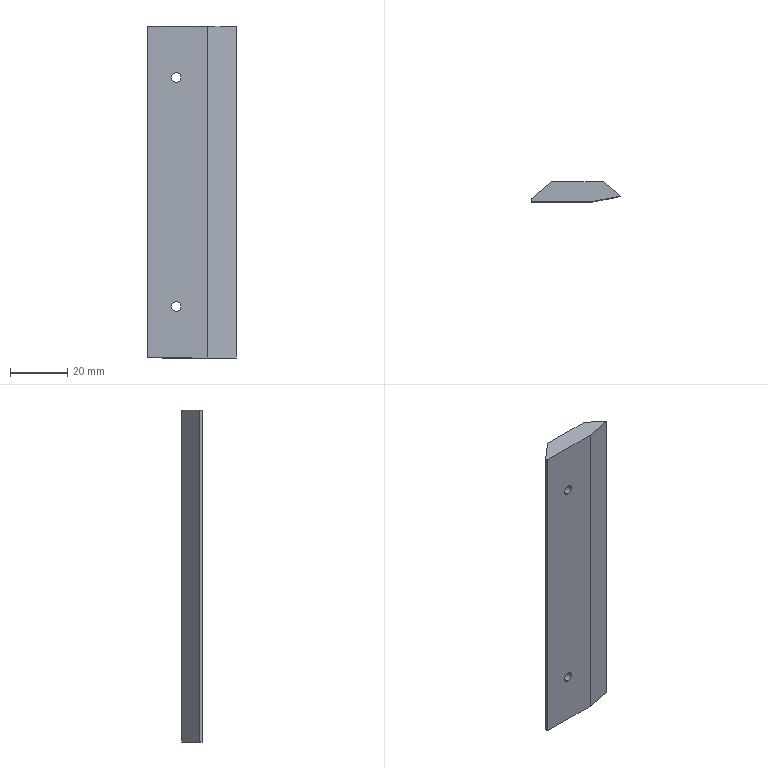Component | SolidWorks | 121.1-1 | 1 solid | 12 faces | box 31 x 7 x 116 mm | volume 19716 mm3 | plane 8 | cylinder 4 | commonest cylinder face diameters 3.3 x4
build123d program:
from build123d import *

# Parameters (mm, degrees)
BOSS_EXTRUDE1_DEPTH   = 58
M4_TAPPED_HOLE1_D     = 3.3
M4_TAPPED_HOLE1_DEPTH = 80
M4_TAPPED_HOLE1_TIP   = 0.9914


with BuildPart() as part:
    # Sketch1 → Boss-Extrude1 (new, symmetric)
    with BuildSketch(Plane.XY):
        Polygon((0, 0), (21, 0), (21, 1), (14, 7), (-4, 7), (-10, 2), align=None)
    extrude(amount=BOSS_EXTRUDE1_DEPTH, both=True)

    # M4 Tapped Hole1
    with Locations(Plane(origin=(0, 7, 0), x_dir=(-1, 0, 0), z_dir=(0, 1, 0))):
        with Locations((-11, 40), (-11, -40)):
            Hole(M4_TAPPED_HOLE1_D / 2, depth=M4_TAPPED_HOLE1_DEPTH)
            with Locations((0, 0, -(M4_TAPPED_HOLE1_DEPTH + M4_TAPPED_HOLE1_TIP / 2))):  # 118° drill point
                Cone(0, M4_TAPPED_HOLE1_D / 2, M4_TAPPED_HOLE1_TIP, mode=Mode.SUBTRACT)


solid = part.part

# Placed as in the assembly
solid = solid.moved(Location((19, 152.5, 0), (-180, 0, 180)))
STEP:
#1=COLOUR_RGB('',0.7922,0.8196,0.9333);
#2=FILL_AREA_STYLE_COLOUR('',#1);
#3=FILL_AREA_STYLE('',(#2));
#4=SURFACE_STYLE_FILL_AREA(#3);
#5=SURFACE_SIDE_STYLE('',(#4));
#6=SURFACE_STYLE_USAGE(.BOTH.,#5);
#7=PRESENTATION_STYLE_ASSIGNMENT((#6));
#8=CARTESIAN_POINT('',(0.315,6.004,-1.51));
#9=VERTEX_POINT('',#8);
#10=CARTESIAN_POINT('',(0.315,6.004,-1.64));
#11=VERTEX_POINT('',#10);
#12=CARTESIAN_POINT('',(0.315,6.004,-1.575));
#13=DIRECTION('',(0.,1.,0.));
#14=DIRECTION('',(-0.,0.,-1.));
#15=AXIS2_PLACEMENT_3D('',#12,#13,#14);
#16=CIRCLE('',#15,0.06496);
#17=EDGE_CURVE('',#9,#11,#16,.T.);
#18=ORIENTED_EDGE('',*,*,#17,.F.);
#19=CARTESIAN_POINT('',(0.315,6.28,-1.51));
#20=VERTEX_POINT('',#19);
#21=CARTESIAN_POINT('',(0.315,6.28,-1.51));
#22=DIRECTION('',(0.,1.,0.));
#23=VECTOR('',#22,39.37);
#24=LINE('',#21,#23);
#25=EDGE_CURVE('',#9,#20,#24,.T.);
#26=ORIENTED_EDGE('',*,*,#25,.T.);
#27=CARTESIAN_POINT('',(0.315,6.28,-1.64));
#28=VERTEX_POINT('',#27);
#29=CARTESIAN_POINT('',(0.315,6.28,-1.575));
#30=DIRECTION('',(0.,1.,0.));
#31=DIRECTION('',(-0.,0.,-1.));
#32=AXIS2_PLACEMENT_3D('',#29,#30,#31);
#33=CIRCLE('',#32,0.06496);
#34=EDGE_CURVE('',#20,#28,#33,.T.);
#35=ORIENTED_EDGE('',*,*,#34,.T.);
#36=CARTESIAN_POINT('',(0.315,6.28,-1.64));
#37=DIRECTION('',(0.,1.,0.));
#38=VECTOR('',#37,39.37);
#39=LINE('',#36,#38);
#40=EDGE_CURVE('',#11,#28,#39,.T.);
#41=ORIENTED_EDGE('',*,*,#40,.F.);
#42=EDGE_LOOP('',(#18,#26,#35,#41));
#43=FACE_OUTER_BOUND('',#42,.T.);
#44=CARTESIAN_POINT('',(0.315,6.28,-1.575));
#45=DIRECTION('',(0.,1.,0.));
#46=DIRECTION('',(-0.,0.,-1.));
#47=AXIS2_PLACEMENT_3D('',#44,#45,#46);
#48=CYLINDRICAL_SURFACE('',#47,0.06496);
#49=ADVANCED_FACE('',(#43),#48,.F.);
#50=CARTESIAN_POINT('',(0.315,6.004,1.64));
#51=VERTEX_POINT('',#50);
#52=CARTESIAN_POINT('',(0.315,6.004,1.51));
#53=VERTEX_POINT('',#52);
#54=CARTESIAN_POINT('',(0.315,6.004,1.575));
#55=DIRECTION('',(0.,1.,0.));
#56=DIRECTION('',(-0.,0.,-1.));
#57=AXIS2_PLACEMENT_3D('',#54,#55,#56);
#58=CIRCLE('',#57,0.06496);
#59=EDGE_CURVE('',#51,#53,#58,.T.);
#60=ORIENTED_EDGE('',*,*,#59,.F.);
#61=CARTESIAN_POINT('',(0.315,6.28,1.64));
#62=VERTEX_POINT('',#61);
#63=CARTESIAN_POINT('',(0.315,6.28,1.64));
#64=DIRECTION('',(0.,1.,0.));
#65=VECTOR('',#64,39.37);
#66=LINE('',#63,#65);
#67=EDGE_CURVE('',#51,#62,#66,.T.);
#68=ORIENTED_EDGE('',*,*,#67,.T.);
#69=CARTESIAN_POINT('',(0.315,6.28,1.51));
#70=VERTEX_POINT('',#69);
#71=CARTESIAN_POINT('',(0.315,6.28,1.575));
#72=DIRECTION('',(0.,1.,0.));
#73=DIRECTION('',(-0.,0.,-1.));
#74=AXIS2_PLACEMENT_3D('',#71,#72,#73);
#75=CIRCLE('',#74,0.06496);
#76=EDGE_CURVE('',#62,#70,#75,.T.);
#77=ORIENTED_EDGE('',*,*,#76,.T.);
#78=CARTESIAN_POINT('',(0.315,6.28,1.51));
#79=DIRECTION('',(0.,1.,0.));
#80=VECTOR('',#79,39.37);
#81=LINE('',#78,#80);
#82=EDGE_CURVE('',#53,#70,#81,.T.);
#83=ORIENTED_EDGE('',*,*,#82,.F.);
#84=EDGE_LOOP('',(#60,#68,#77,#83));
#85=FACE_OUTER_BOUND('',#84,.T.);
#86=CARTESIAN_POINT('',(0.315,6.28,1.575));
#87=DIRECTION('',(0.,1.,0.));
#88=DIRECTION('',(-0.,0.,-1.));
#89=AXIS2_PLACEMENT_3D('',#86,#87,#88);
#90=CYLINDRICAL_SURFACE('',#89,0.06496);
#91=ADVANCED_FACE('',(#85),#90,.F.);
#92=CARTESIAN_POINT('',(1.142,6.083,2.283));
#93=VERTEX_POINT('',#92);
#94=CARTESIAN_POINT('',(0.748,6.004,2.283));
#95=VERTEX_POINT('',#94);
#96=CARTESIAN_POINT('',(1.142,6.083,2.283));
#97=DIRECTION('',(-0.9806,-0.1961,0.));
#98=VECTOR('',#97,39.37);
#99=LINE('',#96,#98);
#100=EDGE_CURVE('',#93,#95,#99,.T.);
#101=ORIENTED_EDGE('',*,*,#100,.T.);
#102=CARTESIAN_POINT('',(0.748,6.004,-2.283));
#103=VERTEX_POINT('',#102);
#104=CARTESIAN_POINT('',(0.748,6.004,-2.283));
#105=DIRECTION('',(0.,-0.,1.));
#106=VECTOR('',#105,39.37);
#107=LINE('',#104,#106);
#108=EDGE_CURVE('',#103,#95,#107,.T.);
#109=ORIENTED_EDGE('',*,*,#108,.F.);
#110=CARTESIAN_POINT('',(1.142,6.083,-2.283));
#111=VERTEX_POINT('',#110);
#112=CARTESIAN_POINT('',(1.142,6.083,-2.283));
#113=DIRECTION('',(-0.9806,-0.1961,0.));
#114=VECTOR('',#113,39.37);
#115=LINE('',#112,#114);
#116=EDGE_CURVE('',#111,#103,#115,.T.);
#117=ORIENTED_EDGE('',*,*,#116,.F.);
#118=CARTESIAN_POINT('',(1.142,6.083,-2.283));
#119=DIRECTION('',(0.,-0.,1.));
#120=VECTOR('',#119,39.37);
#121=LINE('',#118,#120);
#122=EDGE_CURVE('',#111,#93,#121,.T.);
#123=ORIENTED_EDGE('',*,*,#122,.T.);
#124=EDGE_LOOP('',(#101,#109,#117,#123));
#125=FACE_OUTER_BOUND('',#124,.T.);
#126=CARTESIAN_POINT('',(1.142,6.083,-2.283));
#127=DIRECTION('',(-0.1961,0.9806,0.));
#128=DIRECTION('',(0.9806,0.1961,-0.));
#129=AXIS2_PLACEMENT_3D('',#126,#127,#128);
#130=PLANE('',#129);
#131=ADVANCED_FACE('',(#125),#130,.F.);
#132=CARTESIAN_POINT('',(0.315,6.004,-1.575));
#133=DIRECTION('',(0.,1.,0.));
#134=DIRECTION('',(-0.,0.,-1.));
#135=AXIS2_PLACEMENT_3D('',#132,#133,#134);
#136=CIRCLE('',#135,0.06496);
#137=EDGE_CURVE('',#11,#9,#136,.T.);
#138=ORIENTED_EDGE('',*,*,#137,.T.);
#139=ORIENTED_EDGE('',*,*,#17,.T.);
#140=EDGE_LOOP('',(#138,#139));
#141=FACE_BOUND('',#140,.T.);
#142=CARTESIAN_POINT('',(0.315,6.004,1.575));
#143=DIRECTION('',(0.,1.,0.));
#144=DIRECTION('',(-0.,0.,-1.));
#145=AXIS2_PLACEMENT_3D('',#142,#143,#144);
#146=CIRCLE('',#145,0.06496);
#147=EDGE_CURVE('',#53,#51,#146,.T.);
#148=ORIENTED_EDGE('',*,*,#147,.T.);
#149=ORIENTED_EDGE('',*,*,#59,.T.);
#150=EDGE_LOOP('',(#148,#149));
#151=FACE_BOUND('',#150,.T.);
#152=CARTESIAN_POINT('',(-0.07874,6.004,2.283));
#153=VERTEX_POINT('',#152);
#154=CARTESIAN_POINT('',(0.748,6.004,2.283));
#155=DIRECTION('',(-1.,0.,0.));
#156=VECTOR('',#155,39.37);
#157=LINE('',#154,#156);
#158=EDGE_CURVE('',#95,#153,#157,.T.);
#159=ORIENTED_EDGE('',*,*,#158,.T.);
#160=CARTESIAN_POINT('',(-0.07874,6.004,-2.283));
#161=VERTEX_POINT('',#160);
#162=CARTESIAN_POINT('',(-0.07874,6.004,-2.283));
#163=DIRECTION('',(0.,-0.,1.));
#164=VECTOR('',#163,39.37);
#165=LINE('',#162,#164);
#166=EDGE_CURVE('',#161,#153,#165,.T.);
#167=ORIENTED_EDGE('',*,*,#166,.F.);
#168=CARTESIAN_POINT('',(0.748,6.004,-2.283));
#169=DIRECTION('',(-1.,0.,0.));
#170=VECTOR('',#169,39.37);
#171=LINE('',#168,#170);
#172=EDGE_CURVE('',#103,#161,#171,.T.);
#173=ORIENTED_EDGE('',*,*,#172,.F.);
#174=ORIENTED_EDGE('',*,*,#108,.T.);
#175=EDGE_LOOP('',(#159,#167,#173,#174));
#176=FACE_OUTER_BOUND('',#175,.T.);
#177=CARTESIAN_POINT('',(0.748,6.004,-2.283));
#178=DIRECTION('',(0.,1.,0.));
#179=DIRECTION('',(-0.,0.,-1.));
#180=AXIS2_PLACEMENT_3D('',#177,#178,#179);
#181=PLANE('',#180);
#182=ADVANCED_FACE('',(#141,#151,#176),#181,.F.);
#183=CARTESIAN_POINT('',(-0.07874,6.043,2.283));
#184=VERTEX_POINT('',#183);
#185=CARTESIAN_POINT('',(-0.07874,6.004,2.283));
#186=DIRECTION('',(0.,1.,0.));
#187=VECTOR('',#186,39.37);
#188=LINE('',#185,#187);
#189=EDGE_CURVE('',#153,#184,#188,.T.);
#190=ORIENTED_EDGE('',*,*,#189,.T.);
#191=CARTESIAN_POINT('',(-0.07874,6.043,-2.283));
#192=VERTEX_POINT('',#191);
#193=CARTESIAN_POINT('',(-0.07874,6.043,-2.283));
#194=DIRECTION('',(0.,-0.,1.));
#195=VECTOR('',#194,39.37);
#196=LINE('',#193,#195);
#197=EDGE_CURVE('',#192,#184,#196,.T.);
#198=ORIENTED_EDGE('',*,*,#197,.F.);
#199=CARTESIAN_POINT('',(-0.07874,6.004,-2.283));
#200=DIRECTION('',(0.,1.,0.));
#201=VECTOR('',#200,39.37);
#202=LINE('',#199,#201);
#203=EDGE_CURVE('',#161,#192,#202,.T.);
#204=ORIENTED_EDGE('',*,*,#203,.F.);
#205=ORIENTED_EDGE('',*,*,#166,.T.);
#206=EDGE_LOOP('',(#190,#198,#204,#205));
#207=FACE_OUTER_BOUND('',#206,.T.);
#208=CARTESIAN_POINT('',(-0.07874,6.004,-2.283));
#209=DIRECTION('',(1.,-0.,-0.));
#210=DIRECTION('',(-0.,0.,-1.));
#211=AXIS2_PLACEMENT_3D('',#208,#209,#210);
#212=PLANE('',#211);
#213=ADVANCED_FACE('',(#207),#212,.F.);
#214=CARTESIAN_POINT('',(0.1969,6.28,2.283));
#215=VERTEX_POINT('',#214);
#216=CARTESIAN_POINT('',(-0.07874,6.043,2.283));
#217=DIRECTION('',(0.7593,0.6508,-0.));
#218=VECTOR('',#217,39.37);
#219=LINE('',#216,#218);
#220=EDGE_CURVE('',#184,#215,#219,.T.);
#221=ORIENTED_EDGE('',*,*,#220,.T.);
#222=CARTESIAN_POINT('',(0.1969,6.28,-2.283));
#223=VERTEX_POINT('',#222);
#224=CARTESIAN_POINT('',(0.1969,6.28,-2.283));
#225=DIRECTION('',(0.,-0.,1.));
#226=VECTOR('',#225,39.37);
#227=LINE('',#224,#226);
#228=EDGE_CURVE('',#223,#215,#227,.T.);
#229=ORIENTED_EDGE('',*,*,#228,.F.);
#230=CARTESIAN_POINT('',(-0.07874,6.043,-2.283));
#231=DIRECTION('',(0.7593,0.6508,-0.));
#232=VECTOR('',#231,39.37);
#233=LINE('',#230,#232);
#234=EDGE_CURVE('',#192,#223,#233,.T.);
#235=ORIENTED_EDGE('',*,*,#234,.F.);
#236=ORIENTED_EDGE('',*,*,#197,.T.);
#237=EDGE_LOOP('',(#221,#229,#235,#236));
#238=FACE_OUTER_BOUND('',#237,.T.);
#239=CARTESIAN_POINT('',(-0.07874,6.043,-2.283));
#240=DIRECTION('',(0.6508,-0.7593,-0.));
#241=DIRECTION('',(-0.7593,-0.6508,0.));
#242=AXIS2_PLACEMENT_3D('',#239,#240,#241);
#243=PLANE('',#242);
#244=ADVANCED_FACE('',(#238),#243,.F.);
#245=CARTESIAN_POINT('',(0.315,6.28,-1.575));
#246=DIRECTION('',(0.,1.,0.));
#247=DIRECTION('',(-0.,0.,-1.));
#248=AXIS2_PLACEMENT_3D('',#245,#246,#247);
#249=CIRCLE('',#248,0.06496);
#250=EDGE_CURVE('',#28,#20,#249,.T.);
#251=ORIENTED_EDGE('',*,*,#250,.F.);
#252=ORIENTED_EDGE('',*,*,#34,.F.);
#253=EDGE_LOOP('',(#251,#252));
#254=FACE_BOUND('',#253,.T.);
#255=CARTESIAN_POINT('',(0.315,6.28,1.575));
#256=DIRECTION('',(0.,1.,0.));
#257=DIRECTION('',(-0.,0.,-1.));
#258=AXIS2_PLACEMENT_3D('',#255,#256,#257);
#259=CIRCLE('',#258,0.06496);
#260=EDGE_CURVE('',#70,#62,#259,.T.);
#261=ORIENTED_EDGE('',*,*,#260,.F.);
#262=ORIENTED_EDGE('',*,*,#76,.F.);
#263=EDGE_LOOP('',(#261,#262));
#264=FACE_BOUND('',#263,.T.);
#265=CARTESIAN_POINT('',(0.9055,6.28,2.283));
#266=VERTEX_POINT('',#265);
#267=CARTESIAN_POINT('',(0.1969,6.28,2.283));
#268=DIRECTION('',(1.,-0.,-0.));
#269=VECTOR('',#268,39.37);
#270=LINE('',#267,#269);
#271=EDGE_CURVE('',#215,#266,#270,.T.);
#272=ORIENTED_EDGE('',*,*,#271,.T.);
#273=CARTESIAN_POINT('',(0.9055,6.28,-2.283));
#274=VERTEX_POINT('',#273);
#275=CARTESIAN_POINT('',(0.9055,6.28,-2.283));
#276=DIRECTION('',(0.,-0.,1.));
#277=VECTOR('',#276,39.37);
#278=LINE('',#275,#277);
#279=EDGE_CURVE('',#274,#266,#278,.T.);
#280=ORIENTED_EDGE('',*,*,#279,.F.);
#281=CARTESIAN_POINT('',(0.1969,6.28,-2.283));
#282=DIRECTION('',(1.,-0.,-0.));
#283=VECTOR('',#282,39.37);
#284=LINE('',#281,#283);
#285=EDGE_CURVE('',#223,#274,#284,.T.);
#286=ORIENTED_EDGE('',*,*,#285,.F.);
#287=ORIENTED_EDGE('',*,*,#228,.T.);
#288=EDGE_LOOP('',(#272,#280,#286,#287));
#289=FACE_OUTER_BOUND('',#288,.T.);
#290=CARTESIAN_POINT('',(0.1969,6.28,-2.283));
#291=DIRECTION('',(-0.,-1.,-0.));
#292=DIRECTION('',(-1.,0.,0.));
#293=AXIS2_PLACEMENT_3D('',#290,#291,#292);
#294=PLANE('',#293);
#295=ADVANCED_FACE('',(#254,#264,#289),#294,.F.);
#296=CARTESIAN_POINT('',(0.9055,6.28,2.283));
#297=DIRECTION('',(0.7682,-0.6402,-0.));
#298=VECTOR('',#297,39.37);
#299=LINE('',#296,#298);
#300=EDGE_CURVE('',#266,#93,#299,.T.);
#301=ORIENTED_EDGE('',*,*,#300,.T.);
#302=ORIENTED_EDGE('',*,*,#122,.F.);
#303=CARTESIAN_POINT('',(0.9055,6.28,-2.283));
#304=DIRECTION('',(0.7682,-0.6402,-0.));
#305=VECTOR('',#304,39.37);
#306=LINE('',#303,#305);
#307=EDGE_CURVE('',#274,#111,#306,.T.);
#308=ORIENTED_EDGE('',*,*,#307,.F.);
#309=ORIENTED_EDGE('',*,*,#279,.T.);
#310=EDGE_LOOP('',(#301,#302,#308,#309));
#311=FACE_OUTER_BOUND('',#310,.T.);
#312=CARTESIAN_POINT('',(0.9055,6.28,-2.283));
#313=DIRECTION('',(-0.6402,-0.7682,0.));
#314=DIRECTION('',(-0.7682,0.6402,0.));
#315=AXIS2_PLACEMENT_3D('',#312,#313,#314);
#316=PLANE('',#315);
#317=ADVANCED_FACE('',(#311),#316,.F.);
#318=ORIENTED_EDGE('',*,*,#116,.T.);
#319=ORIENTED_EDGE('',*,*,#172,.T.);
#320=ORIENTED_EDGE('',*,*,#203,.T.);
#321=ORIENTED_EDGE('',*,*,#234,.T.);
#322=ORIENTED_EDGE('',*,*,#285,.T.);
#323=ORIENTED_EDGE('',*,*,#307,.T.);
#324=EDGE_LOOP('',(#318,#319,#320,#321,#322,#323));
#325=FACE_OUTER_BOUND('',#324,.T.);
#326=CARTESIAN_POINT('',(-0.07874,5.839,-2.283));
#327=DIRECTION('',(-0.,0.,-1.));
#328=DIRECTION('',(-1.,0.,0.));
#329=AXIS2_PLACEMENT_3D('',#326,#327,#328);
#330=PLANE('',#329);
#331=ADVANCED_FACE('',(#325),#330,.T.);
#332=ORIENTED_EDGE('',*,*,#100,.F.);
#333=ORIENTED_EDGE('',*,*,#300,.F.);
#334=ORIENTED_EDGE('',*,*,#271,.F.);
#335=ORIENTED_EDGE('',*,*,#220,.F.);
#336=ORIENTED_EDGE('',*,*,#189,.F.);
#337=ORIENTED_EDGE('',*,*,#158,.F.);
#338=EDGE_LOOP('',(#332,#333,#334,#335,#336,#337));
#339=FACE_OUTER_BOUND('',#338,.T.);
#340=CARTESIAN_POINT('',(-0.07874,5.839,2.283));
#341=DIRECTION('',(-0.,0.,-1.));
#342=DIRECTION('',(-1.,0.,0.));
#343=AXIS2_PLACEMENT_3D('',#340,#341,#342);
#344=PLANE('',#343);
#345=ADVANCED_FACE('',(#339),#344,.F.);
#346=ORIENTED_EDGE('',*,*,#67,.F.);
#347=ORIENTED_EDGE('',*,*,#147,.F.);
#348=ORIENTED_EDGE('',*,*,#82,.T.);
#349=ORIENTED_EDGE('',*,*,#260,.T.);
#350=EDGE_LOOP('',(#346,#347,#348,#349));
#351=FACE_OUTER_BOUND('',#350,.T.);
#352=CARTESIAN_POINT('',(0.315,6.28,1.575));
#353=DIRECTION('',(0.,1.,0.));
#354=DIRECTION('',(-0.,0.,-1.));
#355=AXIS2_PLACEMENT_3D('',#352,#353,#354);
#356=CYLINDRICAL_SURFACE('',#355,0.06496);
#357=ADVANCED_FACE('',(#351),#356,.F.);
#358=ORIENTED_EDGE('',*,*,#25,.F.);
#359=ORIENTED_EDGE('',*,*,#137,.F.);
#360=ORIENTED_EDGE('',*,*,#40,.T.);
#361=ORIENTED_EDGE('',*,*,#250,.T.);
#362=EDGE_LOOP('',(#358,#359,#360,#361));
#363=FACE_OUTER_BOUND('',#362,.T.);
#364=CARTESIAN_POINT('',(0.315,6.28,-1.575));
#365=DIRECTION('',(0.,1.,0.));
#366=DIRECTION('',(-0.,0.,-1.));
#367=AXIS2_PLACEMENT_3D('',#364,#365,#366);
#368=CYLINDRICAL_SURFACE('',#367,0.06496);
#369=ADVANCED_FACE('',(#363),#368,.F.);
#370=CLOSED_SHELL('',(#49,#91,#131,#182,#213,#244,#295,#317,#331,#345,#357,#369));
#371=MANIFOLD_SOLID_BREP('',#370);
#372=STYLED_ITEM('',(#7),#371);
#373=(LENGTH_UNIT()NAMED_UNIT(*)SI_UNIT($,.METRE.));
#374=LENGTH_MEASURE_WITH_UNIT(LENGTH_MEASURE(0.0254),#373);
#375=DIMENSIONAL_EXPONENTS(1.,0.,0.,0.,0.,0.,0.);
#376=(CONVERSION_BASED_UNIT('',#374)LENGTH_UNIT()NAMED_UNIT(#375));
#377=UNCERTAINTY_MEASURE_WITH_UNIT(LENGTH_MEASURE(0.00001),#376,'','');
#378=(NAMED_UNIT(*)PLANE_ANGLE_UNIT()SI_UNIT($,.RADIAN.));
#379=(NAMED_UNIT(*)SI_UNIT($,.STERADIAN.)SOLID_ANGLE_UNIT());
#380=(GEOMETRIC_REPRESENTATION_CONTEXT(3)GLOBAL_UNCERTAINTY_ASSIGNED_CONTEXT((#377))GLOBAL_UNIT_ASSIGNED_CONTEXT((#376,#378,#379))REPRESENTATION_CONTEXT('',''));
#381=MECHANICAL_DESIGN_GEOMETRIC_PRESENTATION_REPRESENTATION('',(#372),#380);
#382=CARTESIAN_POINT('',(0.,0.,0.));
#383=DIRECTION('',(0.,0.,1.));
#384=DIRECTION('',(1.,0.,0.));
#385=AXIS2_PLACEMENT_3D('',#382,#383,#384);
#386=(LENGTH_UNIT()NAMED_UNIT(*)SI_UNIT($,.METRE.));
#387=LENGTH_MEASURE_WITH_UNIT(LENGTH_MEASURE(0.0254),#386);
#388=DIMENSIONAL_EXPONENTS(1.,0.,0.,0.,0.,0.,0.);
#389=(CONVERSION_BASED_UNIT('',#387)LENGTH_UNIT()NAMED_UNIT(#388));
#390=UNCERTAINTY_MEASURE_WITH_UNIT(LENGTH_MEASURE(0.00001),#389,'','');
#391=(NAMED_UNIT(*)PLANE_ANGLE_UNIT()SI_UNIT($,.RADIAN.));
#392=(NAMED_UNIT(*)SI_UNIT($,.STERADIAN.)SOLID_ANGLE_UNIT());
#393=(GEOMETRIC_REPRESENTATION_CONTEXT(3)GLOBAL_UNCERTAINTY_ASSIGNED_CONTEXT((#390))GLOBAL_UNIT_ASSIGNED_CONTEXT((#389,#391,#392))REPRESENTATION_CONTEXT('',''));
#394=ADVANCED_BREP_SHAPE_REPRESENTATION('',(#371,#385),#393);
#395=PRESENTATION_LAYER_ASSIGNMENT('','',(#372));